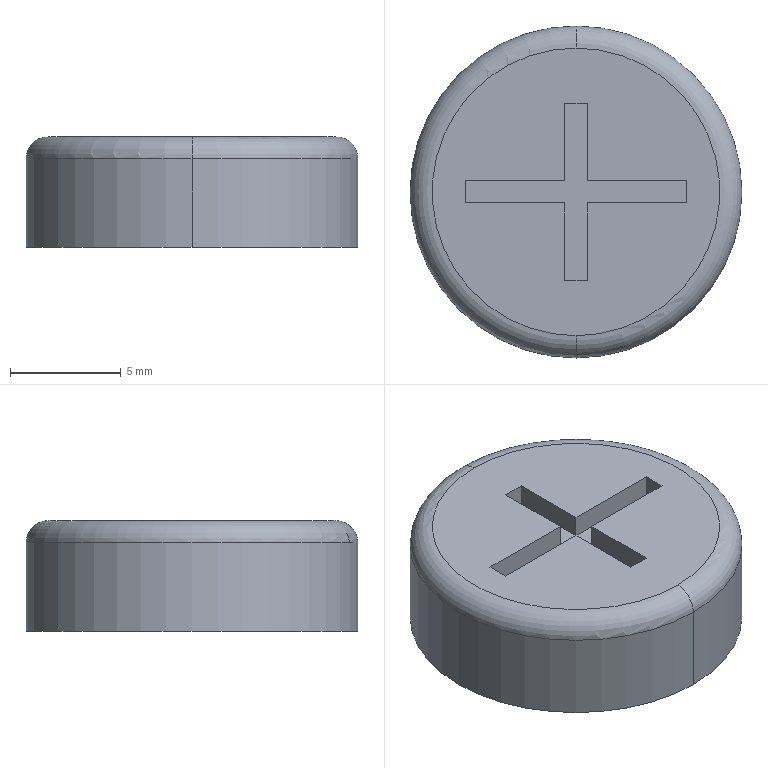Component | SolidWorks | Level-1 | 1 solid | 19 faces | box 15 x 15 x 5 mm | volume 857 mm3 | plane 15 | torus 2 | cylinder 2 | commonest cylinder face diameters 15 x2
STEP:
#1=COLOUR_RGB('',0.7922,0.8196,0.9333);
#2=FILL_AREA_STYLE_COLOUR('',#1);
#3=FILL_AREA_STYLE('',(#2));
#4=SURFACE_STYLE_FILL_AREA(#3);
#5=SURFACE_SIDE_STYLE('',(#4));
#6=SURFACE_STYLE_USAGE(.BOTH.,#5);
#7=PRESENTATION_STYLE_ASSIGNMENT((#6));
#8=CARTESIAN_POINT('',(44.889,53.772,56.593));
#9=VERTEX_POINT('',#8);
#10=CARTESIAN_POINT('',(44.889,53.182,56.593));
#11=VERTEX_POINT('',#10);
#12=CARTESIAN_POINT('',(44.889,53.477,56.593));
#13=DIRECTION('',(0.,0.,-1.));
#14=DIRECTION('',(0.,-1.,0.));
#15=AXIS2_PLACEMENT_3D('',#12,#13,#14);
#16=CIRCLE('',#15,0.2953);
#17=EDGE_CURVE('',#9,#11,#16,.T.);
#18=ORIENTED_EDGE('',*,*,#17,.F.);
#19=CARTESIAN_POINT('',(44.889,53.733,56.632));
#20=VERTEX_POINT('',#19);
#21=CARTESIAN_POINT('',(44.889,53.733,56.593));
#22=DIRECTION('',(1.,-0.,-0.));
#23=DIRECTION('',(0.,1.,0.));
#24=AXIS2_PLACEMENT_3D('',#21,#22,#23);
#25=CIRCLE('',#24,0.03937);
#26=EDGE_CURVE('',#9,#20,#25,.T.);
#27=ORIENTED_EDGE('',*,*,#26,.T.);
#28=CARTESIAN_POINT('',(44.889,53.221,56.632));
#29=VERTEX_POINT('',#28);
#30=CARTESIAN_POINT('',(44.889,53.477,56.632));
#31=DIRECTION('',(0.,-0.,1.));
#32=DIRECTION('',(0.,-1.,0.));
#33=AXIS2_PLACEMENT_3D('',#30,#31,#32);
#34=CIRCLE('',#33,0.2559);
#35=EDGE_CURVE('',#29,#20,#34,.T.);
#36=ORIENTED_EDGE('',*,*,#35,.F.);
#37=CARTESIAN_POINT('',(44.889,53.221,56.593));
#38=DIRECTION('',(-1.,0.,0.));
#39=DIRECTION('',(0.,0.,1.));
#40=AXIS2_PLACEMENT_3D('',#37,#38,#39);
#41=CIRCLE('',#40,0.03937);
#42=EDGE_CURVE('',#11,#29,#41,.T.);
#43=ORIENTED_EDGE('',*,*,#42,.F.);
#44=EDGE_LOOP('',(#18,#27,#36,#43));
#45=FACE_OUTER_BOUND('',#44,.T.);
#46=CARTESIAN_POINT('',(44.889,53.477,56.593));
#47=DIRECTION('',(0.,-0.,1.));
#48=DIRECTION('',(0.,-1.,-0.));
#49=AXIS2_PLACEMENT_3D('',#46,#47,#48);
#50=TOROIDAL_SURFACE('',#49,0.2559,0.03937);
#51=ADVANCED_FACE('',(#45),#50,.T.);
#52=CARTESIAN_POINT('',(44.889,53.182,56.435));
#53=VERTEX_POINT('',#52);
#54=CARTESIAN_POINT('',(44.889,53.772,56.435));
#55=VERTEX_POINT('',#54);
#56=CARTESIAN_POINT('',(44.889,53.477,56.435));
#57=DIRECTION('',(0.,-0.,1.));
#58=DIRECTION('',(0.,-1.,0.));
#59=AXIS2_PLACEMENT_3D('',#56,#57,#58);
#60=CIRCLE('',#59,0.2953);
#61=EDGE_CURVE('',#53,#55,#60,.T.);
#62=ORIENTED_EDGE('',*,*,#61,.T.);
#63=CARTESIAN_POINT('',(44.889,53.772,56.435));
#64=DIRECTION('',(0.,-0.,1.));
#65=VECTOR('',#64,39.37);
#66=LINE('',#63,#65);
#67=EDGE_CURVE('',#55,#9,#66,.T.);
#68=ORIENTED_EDGE('',*,*,#67,.T.);
#69=ORIENTED_EDGE('',*,*,#17,.T.);
#70=CARTESIAN_POINT('',(44.889,53.182,56.435));
#71=DIRECTION('',(0.,-0.,1.));
#72=VECTOR('',#71,39.37);
#73=LINE('',#70,#72);
#74=EDGE_CURVE('',#53,#11,#73,.T.);
#75=ORIENTED_EDGE('',*,*,#74,.F.);
#76=EDGE_LOOP('',(#62,#68,#69,#75));
#77=FACE_OUTER_BOUND('',#76,.T.);
#78=CARTESIAN_POINT('',(44.889,53.477,56.435));
#79=DIRECTION('',(0.,-0.,1.));
#80=DIRECTION('',(0.,-1.,0.));
#81=AXIS2_PLACEMENT_3D('',#78,#79,#80);
#82=CYLINDRICAL_SURFACE('',#81,0.2953);
#83=ADVANCED_FACE('',(#77),#82,.T.);
#84=ORIENTED_EDGE('',*,*,#67,.F.);
#85=CARTESIAN_POINT('',(44.889,53.477,56.435));
#86=DIRECTION('',(0.,-0.,1.));
#87=DIRECTION('',(0.,-1.,0.));
#88=AXIS2_PLACEMENT_3D('',#85,#86,#87);
#89=CIRCLE('',#88,0.2953);
#90=EDGE_CURVE('',#55,#53,#89,.T.);
#91=ORIENTED_EDGE('',*,*,#90,.T.);
#92=ORIENTED_EDGE('',*,*,#74,.T.);
#93=CARTESIAN_POINT('',(44.889,53.477,56.593));
#94=DIRECTION('',(0.,0.,-1.));
#95=DIRECTION('',(0.,-1.,0.));
#96=AXIS2_PLACEMENT_3D('',#93,#94,#95);
#97=CIRCLE('',#96,0.2953);
#98=EDGE_CURVE('',#11,#9,#97,.T.);
#99=ORIENTED_EDGE('',*,*,#98,.T.);
#100=EDGE_LOOP('',(#84,#91,#92,#99));
#101=FACE_OUTER_BOUND('',#100,.T.);
#102=CARTESIAN_POINT('',(44.889,53.477,56.435));
#103=DIRECTION('',(0.,-0.,1.));
#104=DIRECTION('',(0.,-1.,0.));
#105=AXIS2_PLACEMENT_3D('',#102,#103,#104);
#106=CYLINDRICAL_SURFACE('',#105,0.2953);
#107=ADVANCED_FACE('',(#101),#106,.T.);
#108=ORIENTED_EDGE('',*,*,#61,.F.);
#109=ORIENTED_EDGE('',*,*,#90,.F.);
#110=EDGE_LOOP('',(#108,#109));
#111=FACE_OUTER_BOUND('',#110,.T.);
#112=CARTESIAN_POINT('',(44.889,53.477,56.435));
#113=DIRECTION('',(0.,-0.,1.));
#114=DIRECTION('',(0.,-1.,-0.));
#115=AXIS2_PLACEMENT_3D('',#112,#113,#114);
#116=PLANE('',#115);
#117=ADVANCED_FACE('',(#111),#116,.F.);
#118=ORIENTED_EDGE('',*,*,#35,.T.);
#119=CARTESIAN_POINT('',(44.889,53.477,56.632));
#120=DIRECTION('',(0.,-0.,1.));
#121=DIRECTION('',(0.,-1.,0.));
#122=AXIS2_PLACEMENT_3D('',#119,#120,#121);
#123=CIRCLE('',#122,0.2559);
#124=EDGE_CURVE('',#20,#29,#123,.T.);
#125=ORIENTED_EDGE('',*,*,#124,.T.);
#126=EDGE_LOOP('',(#118,#125));
#127=FACE_OUTER_BOUND('',#126,.T.);
#128=CARTESIAN_POINT('',(44.909,53.457,56.632));
#129=VERTEX_POINT('',#128);
#130=CARTESIAN_POINT('',(45.086,53.457,56.632));
#131=VERTEX_POINT('',#130);
#132=CARTESIAN_POINT('',(44.909,53.457,56.632));
#133=DIRECTION('',(1.,-0.,-0.));
#134=VECTOR('',#133,39.37);
#135=LINE('',#132,#134);
#136=EDGE_CURVE('',#129,#131,#135,.T.);
#137=ORIENTED_EDGE('',*,*,#136,.F.);
#138=CARTESIAN_POINT('',(44.909,53.319,56.632));
#139=VERTEX_POINT('',#138);
#140=CARTESIAN_POINT('',(44.909,53.457,56.632));
#141=DIRECTION('',(-0.,1.,0.));
#142=VECTOR('',#141,39.37);
#143=LINE('',#140,#142);
#144=EDGE_CURVE('',#139,#129,#143,.T.);
#145=ORIENTED_EDGE('',*,*,#144,.F.);
#146=CARTESIAN_POINT('',(44.87,53.319,56.632));
#147=VERTEX_POINT('',#146);
#148=CARTESIAN_POINT('',(44.87,53.319,56.632));
#149=DIRECTION('',(1.,0.,0.));
#150=VECTOR('',#149,39.37);
#151=LINE('',#148,#150);
#152=EDGE_CURVE('',#147,#139,#151,.T.);
#153=ORIENTED_EDGE('',*,*,#152,.F.);
#154=CARTESIAN_POINT('',(44.87,53.457,56.632));
#155=VERTEX_POINT('',#154);
#156=CARTESIAN_POINT('',(44.87,53.457,56.632));
#157=DIRECTION('',(0.,-1.,-0.));
#158=VECTOR('',#157,39.37);
#159=LINE('',#156,#158);
#160=EDGE_CURVE('',#155,#147,#159,.T.);
#161=ORIENTED_EDGE('',*,*,#160,.F.);
#162=CARTESIAN_POINT('',(44.692,53.457,56.632));
#163=VERTEX_POINT('',#162);
#164=CARTESIAN_POINT('',(44.692,53.457,56.632));
#165=DIRECTION('',(1.,-0.,-0.));
#166=VECTOR('',#165,39.37);
#167=LINE('',#164,#166);
#168=EDGE_CURVE('',#163,#155,#167,.T.);
#169=ORIENTED_EDGE('',*,*,#168,.F.);
#170=CARTESIAN_POINT('',(44.692,53.497,56.632));
#171=VERTEX_POINT('',#170);
#172=CARTESIAN_POINT('',(44.692,53.497,56.632));
#173=DIRECTION('',(0.,-1.,-0.));
#174=VECTOR('',#173,39.37);
#175=LINE('',#172,#174);
#176=EDGE_CURVE('',#171,#163,#175,.T.);
#177=ORIENTED_EDGE('',*,*,#176,.F.);
#178=CARTESIAN_POINT('',(44.87,53.497,56.632));
#179=VERTEX_POINT('',#178);
#180=CARTESIAN_POINT('',(44.692,53.497,56.632));
#181=DIRECTION('',(-1.,0.,0.));
#182=VECTOR('',#181,39.37);
#183=LINE('',#180,#182);
#184=EDGE_CURVE('',#179,#171,#183,.T.);
#185=ORIENTED_EDGE('',*,*,#184,.F.);
#186=CARTESIAN_POINT('',(44.87,53.634,56.632));
#187=VERTEX_POINT('',#186);
#188=CARTESIAN_POINT('',(44.87,53.634,56.632));
#189=DIRECTION('',(0.,-1.,-0.));
#190=VECTOR('',#189,39.37);
#191=LINE('',#188,#190);
#192=EDGE_CURVE('',#187,#179,#191,.T.);
#193=ORIENTED_EDGE('',*,*,#192,.F.);
#194=CARTESIAN_POINT('',(44.909,53.634,56.632));
#195=VERTEX_POINT('',#194);
#196=CARTESIAN_POINT('',(44.87,53.634,56.632));
#197=DIRECTION('',(-1.,0.,0.));
#198=VECTOR('',#197,39.37);
#199=LINE('',#196,#198);
#200=EDGE_CURVE('',#195,#187,#199,.T.);
#201=ORIENTED_EDGE('',*,*,#200,.F.);
#202=CARTESIAN_POINT('',(44.909,53.497,56.632));
#203=VERTEX_POINT('',#202);
#204=CARTESIAN_POINT('',(44.909,53.634,56.632));
#205=DIRECTION('',(-0.,1.,0.));
#206=VECTOR('',#205,39.37);
#207=LINE('',#204,#206);
#208=EDGE_CURVE('',#203,#195,#207,.T.);
#209=ORIENTED_EDGE('',*,*,#208,.F.);
#210=CARTESIAN_POINT('',(45.086,53.497,56.632));
#211=VERTEX_POINT('',#210);
#212=CARTESIAN_POINT('',(44.909,53.497,56.632));
#213=DIRECTION('',(-1.,-0.,-0.));
#214=VECTOR('',#213,39.37);
#215=LINE('',#212,#214);
#216=EDGE_CURVE('',#211,#203,#215,.T.);
#217=ORIENTED_EDGE('',*,*,#216,.F.);
#218=CARTESIAN_POINT('',(45.086,53.497,56.632));
#219=DIRECTION('',(0.,1.,0.));
#220=VECTOR('',#219,39.37);
#221=LINE('',#218,#220);
#222=EDGE_CURVE('',#131,#211,#221,.T.);
#223=ORIENTED_EDGE('',*,*,#222,.F.);
#224=EDGE_LOOP('',(#137,#145,#153,#161,#169,#177,#185,#193,#201,#209,#217,#223));
#225=FACE_BOUND('',#224,.T.);
#226=CARTESIAN_POINT('',(44.889,53.477,56.632));
#227=DIRECTION('',(0.,-0.,1.));
#228=DIRECTION('',(0.,-1.,-0.));
#229=AXIS2_PLACEMENT_3D('',#226,#227,#228);
#230=PLANE('',#229);
#231=ADVANCED_FACE('',(#127,#225),#230,.T.);
#232=ORIENTED_EDGE('',*,*,#136,.T.);
#233=CARTESIAN_POINT('',(45.086,53.457,56.593));
#234=VERTEX_POINT('',#233);
#235=CARTESIAN_POINT('',(45.086,53.457,56.593));
#236=DIRECTION('',(0.,-0.,1.));
#237=VECTOR('',#236,39.37);
#238=LINE('',#235,#237);
#239=EDGE_CURVE('',#234,#131,#238,.T.);
#240=ORIENTED_EDGE('',*,*,#239,.F.);
#241=CARTESIAN_POINT('',(44.909,53.457,56.593));
#242=VERTEX_POINT('',#241);
#243=CARTESIAN_POINT('',(44.909,53.457,56.593));
#244=DIRECTION('',(1.,-0.,-0.));
#245=VECTOR('',#244,39.37);
#246=LINE('',#243,#245);
#247=EDGE_CURVE('',#242,#234,#246,.T.);
#248=ORIENTED_EDGE('',*,*,#247,.F.);
#249=CARTESIAN_POINT('',(44.909,53.457,56.593));
#250=DIRECTION('',(0.,-0.,1.));
#251=VECTOR('',#250,39.37);
#252=LINE('',#249,#251);
#253=EDGE_CURVE('',#242,#129,#252,.T.);
#254=ORIENTED_EDGE('',*,*,#253,.T.);
#255=EDGE_LOOP('',(#232,#240,#248,#254));
#256=FACE_OUTER_BOUND('',#255,.T.);
#257=CARTESIAN_POINT('',(44.909,53.457,56.593));
#258=DIRECTION('',(-0.,-1.,-0.));
#259=DIRECTION('',(1.,-0.,-0.));
#260=AXIS2_PLACEMENT_3D('',#257,#258,#259);
#261=PLANE('',#260);
#262=ADVANCED_FACE('',(#256),#261,.F.);
#263=ORIENTED_EDGE('',*,*,#144,.T.);
#264=ORIENTED_EDGE('',*,*,#253,.F.);
#265=CARTESIAN_POINT('',(44.909,53.319,56.593));
#266=VERTEX_POINT('',#265);
#267=CARTESIAN_POINT('',(44.909,53.457,56.593));
#268=DIRECTION('',(-0.,1.,0.));
#269=VECTOR('',#268,39.37);
#270=LINE('',#267,#269);
#271=EDGE_CURVE('',#266,#242,#270,.T.);
#272=ORIENTED_EDGE('',*,*,#271,.F.);
#273=CARTESIAN_POINT('',(44.909,53.319,56.593));
#274=DIRECTION('',(0.,-0.,1.));
#275=VECTOR('',#274,39.37);
#276=LINE('',#273,#275);
#277=EDGE_CURVE('',#266,#139,#276,.T.);
#278=ORIENTED_EDGE('',*,*,#277,.T.);
#279=EDGE_LOOP('',(#263,#264,#272,#278));
#280=FACE_OUTER_BOUND('',#279,.T.);
#281=CARTESIAN_POINT('',(44.909,53.457,56.593));
#282=DIRECTION('',(1.,0.,0.));
#283=DIRECTION('',(-0.,1.,0.));
#284=AXIS2_PLACEMENT_3D('',#281,#282,#283);
#285=PLANE('',#284);
#286=ADVANCED_FACE('',(#280),#285,.F.);
#287=ORIENTED_EDGE('',*,*,#152,.T.);
#288=ORIENTED_EDGE('',*,*,#277,.F.);
#289=CARTESIAN_POINT('',(44.87,53.319,56.593));
#290=VERTEX_POINT('',#289);
#291=CARTESIAN_POINT('',(44.87,53.319,56.593));
#292=DIRECTION('',(1.,0.,0.));
#293=VECTOR('',#292,39.37);
#294=LINE('',#291,#293);
#295=EDGE_CURVE('',#290,#266,#294,.T.);
#296=ORIENTED_EDGE('',*,*,#295,.F.);
#297=CARTESIAN_POINT('',(44.87,53.319,56.593));
#298=DIRECTION('',(0.,-0.,1.));
#299=VECTOR('',#298,39.37);
#300=LINE('',#297,#299);
#301=EDGE_CURVE('',#290,#147,#300,.T.);
#302=ORIENTED_EDGE('',*,*,#301,.T.);
#303=EDGE_LOOP('',(#287,#288,#296,#302));
#304=FACE_OUTER_BOUND('',#303,.T.);
#305=CARTESIAN_POINT('',(44.87,53.319,56.593));
#306=DIRECTION('',(0.,-1.,-0.));
#307=DIRECTION('',(1.,0.,0.));
#308=AXIS2_PLACEMENT_3D('',#305,#306,#307);
#309=PLANE('',#308);
#310=ADVANCED_FACE('',(#304),#309,.F.);
#311=ORIENTED_EDGE('',*,*,#160,.T.);
#312=ORIENTED_EDGE('',*,*,#301,.F.);
#313=CARTESIAN_POINT('',(44.87,53.457,56.593));
#314=VERTEX_POINT('',#313);
#315=CARTESIAN_POINT('',(44.87,53.457,56.593));
#316=DIRECTION('',(0.,-1.,-0.));
#317=VECTOR('',#316,39.37);
#318=LINE('',#315,#317);
#319=EDGE_CURVE('',#314,#290,#318,.T.);
#320=ORIENTED_EDGE('',*,*,#319,.F.);
#321=CARTESIAN_POINT('',(44.87,53.457,56.593));
#322=DIRECTION('',(0.,-0.,1.));
#323=VECTOR('',#322,39.37);
#324=LINE('',#321,#323);
#325=EDGE_CURVE('',#314,#155,#324,.T.);
#326=ORIENTED_EDGE('',*,*,#325,.T.);
#327=EDGE_LOOP('',(#311,#312,#320,#326));
#328=FACE_OUTER_BOUND('',#327,.T.);
#329=CARTESIAN_POINT('',(44.87,53.457,56.593));
#330=DIRECTION('',(-1.,-0.,-0.));
#331=DIRECTION('',(0.,-1.,-0.));
#332=AXIS2_PLACEMENT_3D('',#329,#330,#331);
#333=PLANE('',#332);
#334=ADVANCED_FACE('',(#328),#333,.F.);
#335=ORIENTED_EDGE('',*,*,#168,.T.);
#336=ORIENTED_EDGE('',*,*,#325,.F.);
#337=CARTESIAN_POINT('',(44.692,53.457,56.593));
#338=VERTEX_POINT('',#337);
#339=CARTESIAN_POINT('',(44.692,53.457,56.593));
#340=DIRECTION('',(1.,-0.,-0.));
#341=VECTOR('',#340,39.37);
#342=LINE('',#339,#341);
#343=EDGE_CURVE('',#338,#314,#342,.T.);
#344=ORIENTED_EDGE('',*,*,#343,.F.);
#345=CARTESIAN_POINT('',(44.692,53.457,56.593));
#346=DIRECTION('',(0.,-0.,1.));
#347=VECTOR('',#346,39.37);
#348=LINE('',#345,#347);
#349=EDGE_CURVE('',#338,#163,#348,.T.);
#350=ORIENTED_EDGE('',*,*,#349,.T.);
#351=EDGE_LOOP('',(#335,#336,#344,#350));
#352=FACE_OUTER_BOUND('',#351,.T.);
#353=CARTESIAN_POINT('',(44.692,53.457,56.593));
#354=DIRECTION('',(-0.,-1.,-0.));
#355=DIRECTION('',(1.,-0.,-0.));
#356=AXIS2_PLACEMENT_3D('',#353,#354,#355);
#357=PLANE('',#356);
#358=ADVANCED_FACE('',(#352),#357,.F.);
#359=ORIENTED_EDGE('',*,*,#176,.T.);
#360=ORIENTED_EDGE('',*,*,#349,.F.);
#361=CARTESIAN_POINT('',(44.692,53.497,56.593));
#362=VERTEX_POINT('',#361);
#363=CARTESIAN_POINT('',(44.692,53.497,56.593));
#364=DIRECTION('',(0.,-1.,-0.));
#365=VECTOR('',#364,39.37);
#366=LINE('',#363,#365);
#367=EDGE_CURVE('',#362,#338,#366,.T.);
#368=ORIENTED_EDGE('',*,*,#367,.F.);
#369=CARTESIAN_POINT('',(44.692,53.497,56.593));
#370=DIRECTION('',(0.,-0.,1.));
#371=VECTOR('',#370,39.37);
#372=LINE('',#369,#371);
#373=EDGE_CURVE('',#362,#171,#372,.T.);
#374=ORIENTED_EDGE('',*,*,#373,.T.);
#375=EDGE_LOOP('',(#359,#360,#368,#374));
#376=FACE_OUTER_BOUND('',#375,.T.);
#377=CARTESIAN_POINT('',(44.692,53.497,56.593));
#378=DIRECTION('',(-1.,0.,0.));
#379=DIRECTION('',(0.,-1.,-0.));
#380=AXIS2_PLACEMENT_3D('',#377,#378,#379);
#381=PLANE('',#380);
#382=ADVANCED_FACE('',(#376),#381,.F.);
#383=ORIENTED_EDGE('',*,*,#184,.T.);
#384=ORIENTED_EDGE('',*,*,#373,.F.);
#385=CARTESIAN_POINT('',(44.87,53.497,56.593));
#386=VERTEX_POINT('',#385);
#387=CARTESIAN_POINT('',(44.692,53.497,56.593));
#388=DIRECTION('',(-1.,0.,0.));
#389=VECTOR('',#388,39.37);
#390=LINE('',#387,#389);
#391=EDGE_CURVE('',#386,#362,#390,.T.);
#392=ORIENTED_EDGE('',*,*,#391,.F.);
#393=CARTESIAN_POINT('',(44.87,53.497,56.593));
#394=DIRECTION('',(0.,-0.,1.));
#395=VECTOR('',#394,39.37);
#396=LINE('',#393,#395);
#397=EDGE_CURVE('',#386,#179,#396,.T.);
#398=ORIENTED_EDGE('',*,*,#397,.T.);
#399=EDGE_LOOP('',(#383,#384,#392,#398));
#400=FACE_OUTER_BOUND('',#399,.T.);
#401=CARTESIAN_POINT('',(44.692,53.497,56.593));
#402=DIRECTION('',(0.,1.,0.));
#403=DIRECTION('',(-1.,0.,0.));
#404=AXIS2_PLACEMENT_3D('',#401,#402,#403);
#405=PLANE('',#404);
#406=ADVANCED_FACE('',(#400),#405,.F.);
#407=ORIENTED_EDGE('',*,*,#192,.T.);
#408=ORIENTED_EDGE('',*,*,#397,.F.);
#409=CARTESIAN_POINT('',(44.87,53.634,56.593));
#410=VERTEX_POINT('',#409);
#411=CARTESIAN_POINT('',(44.87,53.634,56.593));
#412=DIRECTION('',(0.,-1.,-0.));
#413=VECTOR('',#412,39.37);
#414=LINE('',#411,#413);
#415=EDGE_CURVE('',#410,#386,#414,.T.);
#416=ORIENTED_EDGE('',*,*,#415,.F.);
#417=CARTESIAN_POINT('',(44.87,53.634,56.593));
#418=DIRECTION('',(0.,-0.,1.));
#419=VECTOR('',#418,39.37);
#420=LINE('',#417,#419);
#421=EDGE_CURVE('',#410,#187,#420,.T.);
#422=ORIENTED_EDGE('',*,*,#421,.T.);
#423=EDGE_LOOP('',(#407,#408,#416,#422));
#424=FACE_OUTER_BOUND('',#423,.T.);
#425=CARTESIAN_POINT('',(44.87,53.634,56.593));
#426=DIRECTION('',(-1.,-0.,-0.));
#427=DIRECTION('',(0.,-1.,-0.));
#428=AXIS2_PLACEMENT_3D('',#425,#426,#427);
#429=PLANE('',#428);
#430=ADVANCED_FACE('',(#424),#429,.F.);
#431=ORIENTED_EDGE('',*,*,#200,.T.);
#432=ORIENTED_EDGE('',*,*,#421,.F.);
#433=CARTESIAN_POINT('',(44.909,53.634,56.593));
#434=VERTEX_POINT('',#433);
#435=CARTESIAN_POINT('',(44.87,53.634,56.593));
#436=DIRECTION('',(-1.,0.,0.));
#437=VECTOR('',#436,39.37);
#438=LINE('',#435,#437);
#439=EDGE_CURVE('',#434,#410,#438,.T.);
#440=ORIENTED_EDGE('',*,*,#439,.F.);
#441=CARTESIAN_POINT('',(44.909,53.634,56.593));
#442=DIRECTION('',(0.,-0.,1.));
#443=VECTOR('',#442,39.37);
#444=LINE('',#441,#443);
#445=EDGE_CURVE('',#434,#195,#444,.T.);
#446=ORIENTED_EDGE('',*,*,#445,.T.);
#447=EDGE_LOOP('',(#431,#432,#440,#446));
#448=FACE_OUTER_BOUND('',#447,.T.);
#449=CARTESIAN_POINT('',(44.87,53.634,56.593));
#450=DIRECTION('',(0.,1.,0.));
#451=DIRECTION('',(-1.,0.,0.));
#452=AXIS2_PLACEMENT_3D('',#449,#450,#451);
#453=PLANE('',#452);
#454=ADVANCED_FACE('',(#448),#453,.F.);
#455=ORIENTED_EDGE('',*,*,#208,.T.);
#456=ORIENTED_EDGE('',*,*,#445,.F.);
#457=CARTESIAN_POINT('',(44.909,53.497,56.593));
#458=VERTEX_POINT('',#457);
#459=CARTESIAN_POINT('',(44.909,53.634,56.593));
#460=DIRECTION('',(-0.,1.,0.));
#461=VECTOR('',#460,39.37);
#462=LINE('',#459,#461);
#463=EDGE_CURVE('',#458,#434,#462,.T.);
#464=ORIENTED_EDGE('',*,*,#463,.F.);
#465=CARTESIAN_POINT('',(44.909,53.497,56.593));
#466=DIRECTION('',(0.,-0.,1.));
#467=VECTOR('',#466,39.37);
#468=LINE('',#465,#467);
#469=EDGE_CURVE('',#458,#203,#468,.T.);
#470=ORIENTED_EDGE('',*,*,#469,.T.);
#471=EDGE_LOOP('',(#455,#456,#464,#470));
#472=FACE_OUTER_BOUND('',#471,.T.);
#473=CARTESIAN_POINT('',(44.909,53.634,56.593));
#474=DIRECTION('',(1.,0.,0.));
#475=DIRECTION('',(-0.,1.,0.));
#476=AXIS2_PLACEMENT_3D('',#473,#474,#475);
#477=PLANE('',#476);
#478=ADVANCED_FACE('',(#472),#477,.F.);
#479=ORIENTED_EDGE('',*,*,#216,.T.);
#480=ORIENTED_EDGE('',*,*,#469,.F.);
#481=CARTESIAN_POINT('',(45.086,53.497,56.593));
#482=VERTEX_POINT('',#481);
#483=CARTESIAN_POINT('',(44.909,53.497,56.593));
#484=DIRECTION('',(-1.,-0.,-0.));
#485=VECTOR('',#484,39.37);
#486=LINE('',#483,#485);
#487=EDGE_CURVE('',#482,#458,#486,.T.);
#488=ORIENTED_EDGE('',*,*,#487,.F.);
#489=CARTESIAN_POINT('',(45.086,53.497,56.593));
#490=DIRECTION('',(0.,-0.,1.));
#491=VECTOR('',#490,39.37);
#492=LINE('',#489,#491);
#493=EDGE_CURVE('',#482,#211,#492,.T.);
#494=ORIENTED_EDGE('',*,*,#493,.T.);
#495=EDGE_LOOP('',(#479,#480,#488,#494));
#496=FACE_OUTER_BOUND('',#495,.T.);
#497=CARTESIAN_POINT('',(44.909,53.497,56.593));
#498=DIRECTION('',(-0.,1.,0.));
#499=DIRECTION('',(-1.,-0.,-0.));
#500=AXIS2_PLACEMENT_3D('',#497,#498,#499);
#501=PLANE('',#500);
#502=ADVANCED_FACE('',(#496),#501,.F.);
#503=ORIENTED_EDGE('',*,*,#222,.T.);
#504=ORIENTED_EDGE('',*,*,#493,.F.);
#505=CARTESIAN_POINT('',(45.086,53.497,56.593));
#506=DIRECTION('',(0.,1.,0.));
#507=VECTOR('',#506,39.37);
#508=LINE('',#505,#507);
#509=EDGE_CURVE('',#234,#482,#508,.T.);
#510=ORIENTED_EDGE('',*,*,#509,.F.);
#511=ORIENTED_EDGE('',*,*,#239,.T.);
#512=EDGE_LOOP('',(#503,#504,#510,#511));
#513=FACE_OUTER_BOUND('',#512,.T.);
#514=CARTESIAN_POINT('',(45.086,53.497,56.593));
#515=DIRECTION('',(1.,0.,0.));
#516=DIRECTION('',(0.,1.,0.));
#517=AXIS2_PLACEMENT_3D('',#514,#515,#516);
#518=PLANE('',#517);
#519=ADVANCED_FACE('',(#513),#518,.F.);
#520=ORIENTED_EDGE('',*,*,#247,.T.);
#521=ORIENTED_EDGE('',*,*,#509,.T.);
#522=ORIENTED_EDGE('',*,*,#487,.T.);
#523=ORIENTED_EDGE('',*,*,#463,.T.);
#524=ORIENTED_EDGE('',*,*,#439,.T.);
#525=ORIENTED_EDGE('',*,*,#415,.T.);
#526=ORIENTED_EDGE('',*,*,#391,.T.);
#527=ORIENTED_EDGE('',*,*,#367,.T.);
#528=ORIENTED_EDGE('',*,*,#343,.T.);
#529=ORIENTED_EDGE('',*,*,#319,.T.);
#530=ORIENTED_EDGE('',*,*,#295,.T.);
#531=ORIENTED_EDGE('',*,*,#271,.T.);
#532=EDGE_LOOP('',(#520,#521,#522,#523,#524,#525,#526,#527,#528,#529,#530,#531));
#533=FACE_OUTER_BOUND('',#532,.T.);
#534=CARTESIAN_POINT('',(44.889,53.477,56.593));
#535=DIRECTION('',(0.,0.,-1.));
#536=DIRECTION('',(0.,1.,0.));
#537=AXIS2_PLACEMENT_3D('',#534,#535,#536);
#538=PLANE('',#537);
#539=ADVANCED_FACE('',(#533),#538,.F.);
#540=ORIENTED_EDGE('',*,*,#26,.F.);
#541=ORIENTED_EDGE('',*,*,#98,.F.);
#542=ORIENTED_EDGE('',*,*,#42,.T.);
#543=ORIENTED_EDGE('',*,*,#124,.F.);
#544=EDGE_LOOP('',(#540,#541,#542,#543));
#545=FACE_OUTER_BOUND('',#544,.T.);
#546=CARTESIAN_POINT('',(44.889,53.477,56.593));
#547=DIRECTION('',(0.,-0.,1.));
#548=DIRECTION('',(0.,-1.,-0.));
#549=AXIS2_PLACEMENT_3D('',#546,#547,#548);
#550=TOROIDAL_SURFACE('',#549,0.2559,0.03937);
#551=ADVANCED_FACE('',(#545),#550,.T.);
#552=CLOSED_SHELL('',(#51,#83,#107,#117,#231,#262,#286,#310,#334,#358,#382,#406,#430,#454,#478,#502,#519,#539,#551));
#553=MANIFOLD_SOLID_BREP('',#552);
#554=STYLED_ITEM('',(#7),#553);
#555=(LENGTH_UNIT()NAMED_UNIT(*)SI_UNIT($,.METRE.));
#556=LENGTH_MEASURE_WITH_UNIT(LENGTH_MEASURE(0.0254),#555);
#557=DIMENSIONAL_EXPONENTS(1.,0.,0.,0.,0.,0.,0.);
#558=(CONVERSION_BASED_UNIT('',#556)LENGTH_UNIT()NAMED_UNIT(#557));
#559=UNCERTAINTY_MEASURE_WITH_UNIT(LENGTH_MEASURE(0.00001),#558,'','');
#560=(NAMED_UNIT(*)PLANE_ANGLE_UNIT()SI_UNIT($,.RADIAN.));
#561=(NAMED_UNIT(*)SI_UNIT($,.STERADIAN.)SOLID_ANGLE_UNIT());
#562=(GEOMETRIC_REPRESENTATION_CONTEXT(3)GLOBAL_UNCERTAINTY_ASSIGNED_CONTEXT((#559))GLOBAL_UNIT_ASSIGNED_CONTEXT((#558,#560,#561))REPRESENTATION_CONTEXT('',''));
#563=MECHANICAL_DESIGN_GEOMETRIC_PRESENTATION_REPRESENTATION('',(#554),#562);
#564=PRESENTATION_LAYER_ASSIGNMENT('','',(#554));
#565=CARTESIAN_POINT('',(0.,0.,0.));
#566=DIRECTION('',(0.,0.,1.));
#567=DIRECTION('',(1.,0.,0.));
#568=AXIS2_PLACEMENT_3D('',#565,#566,#567);
#569=(LENGTH_UNIT()NAMED_UNIT(*)SI_UNIT($,.METRE.));
#570=LENGTH_MEASURE_WITH_UNIT(LENGTH_MEASURE(0.0254),#569);
#571=DIMENSIONAL_EXPONENTS(1.,0.,0.,0.,0.,0.,0.);
#572=(CONVERSION_BASED_UNIT('',#570)LENGTH_UNIT()NAMED_UNIT(#571));
#573=UNCERTAINTY_MEASURE_WITH_UNIT(LENGTH_MEASURE(0.00001),#572,'','');
#574=(NAMED_UNIT(*)PLANE_ANGLE_UNIT()SI_UNIT($,.RADIAN.));
#575=(NAMED_UNIT(*)SI_UNIT($,.STERADIAN.)SOLID_ANGLE_UNIT());
#576=(GEOMETRIC_REPRESENTATION_CONTEXT(3)GLOBAL_UNCERTAINTY_ASSIGNED_CONTEXT((#573))GLOBAL_UNIT_ASSIGNED_CONTEXT((#572,#574,#575))REPRESENTATION_CONTEXT('',''));
#577=ADVANCED_BREP_SHAPE_REPRESENTATION('',(#553,#568),#576);